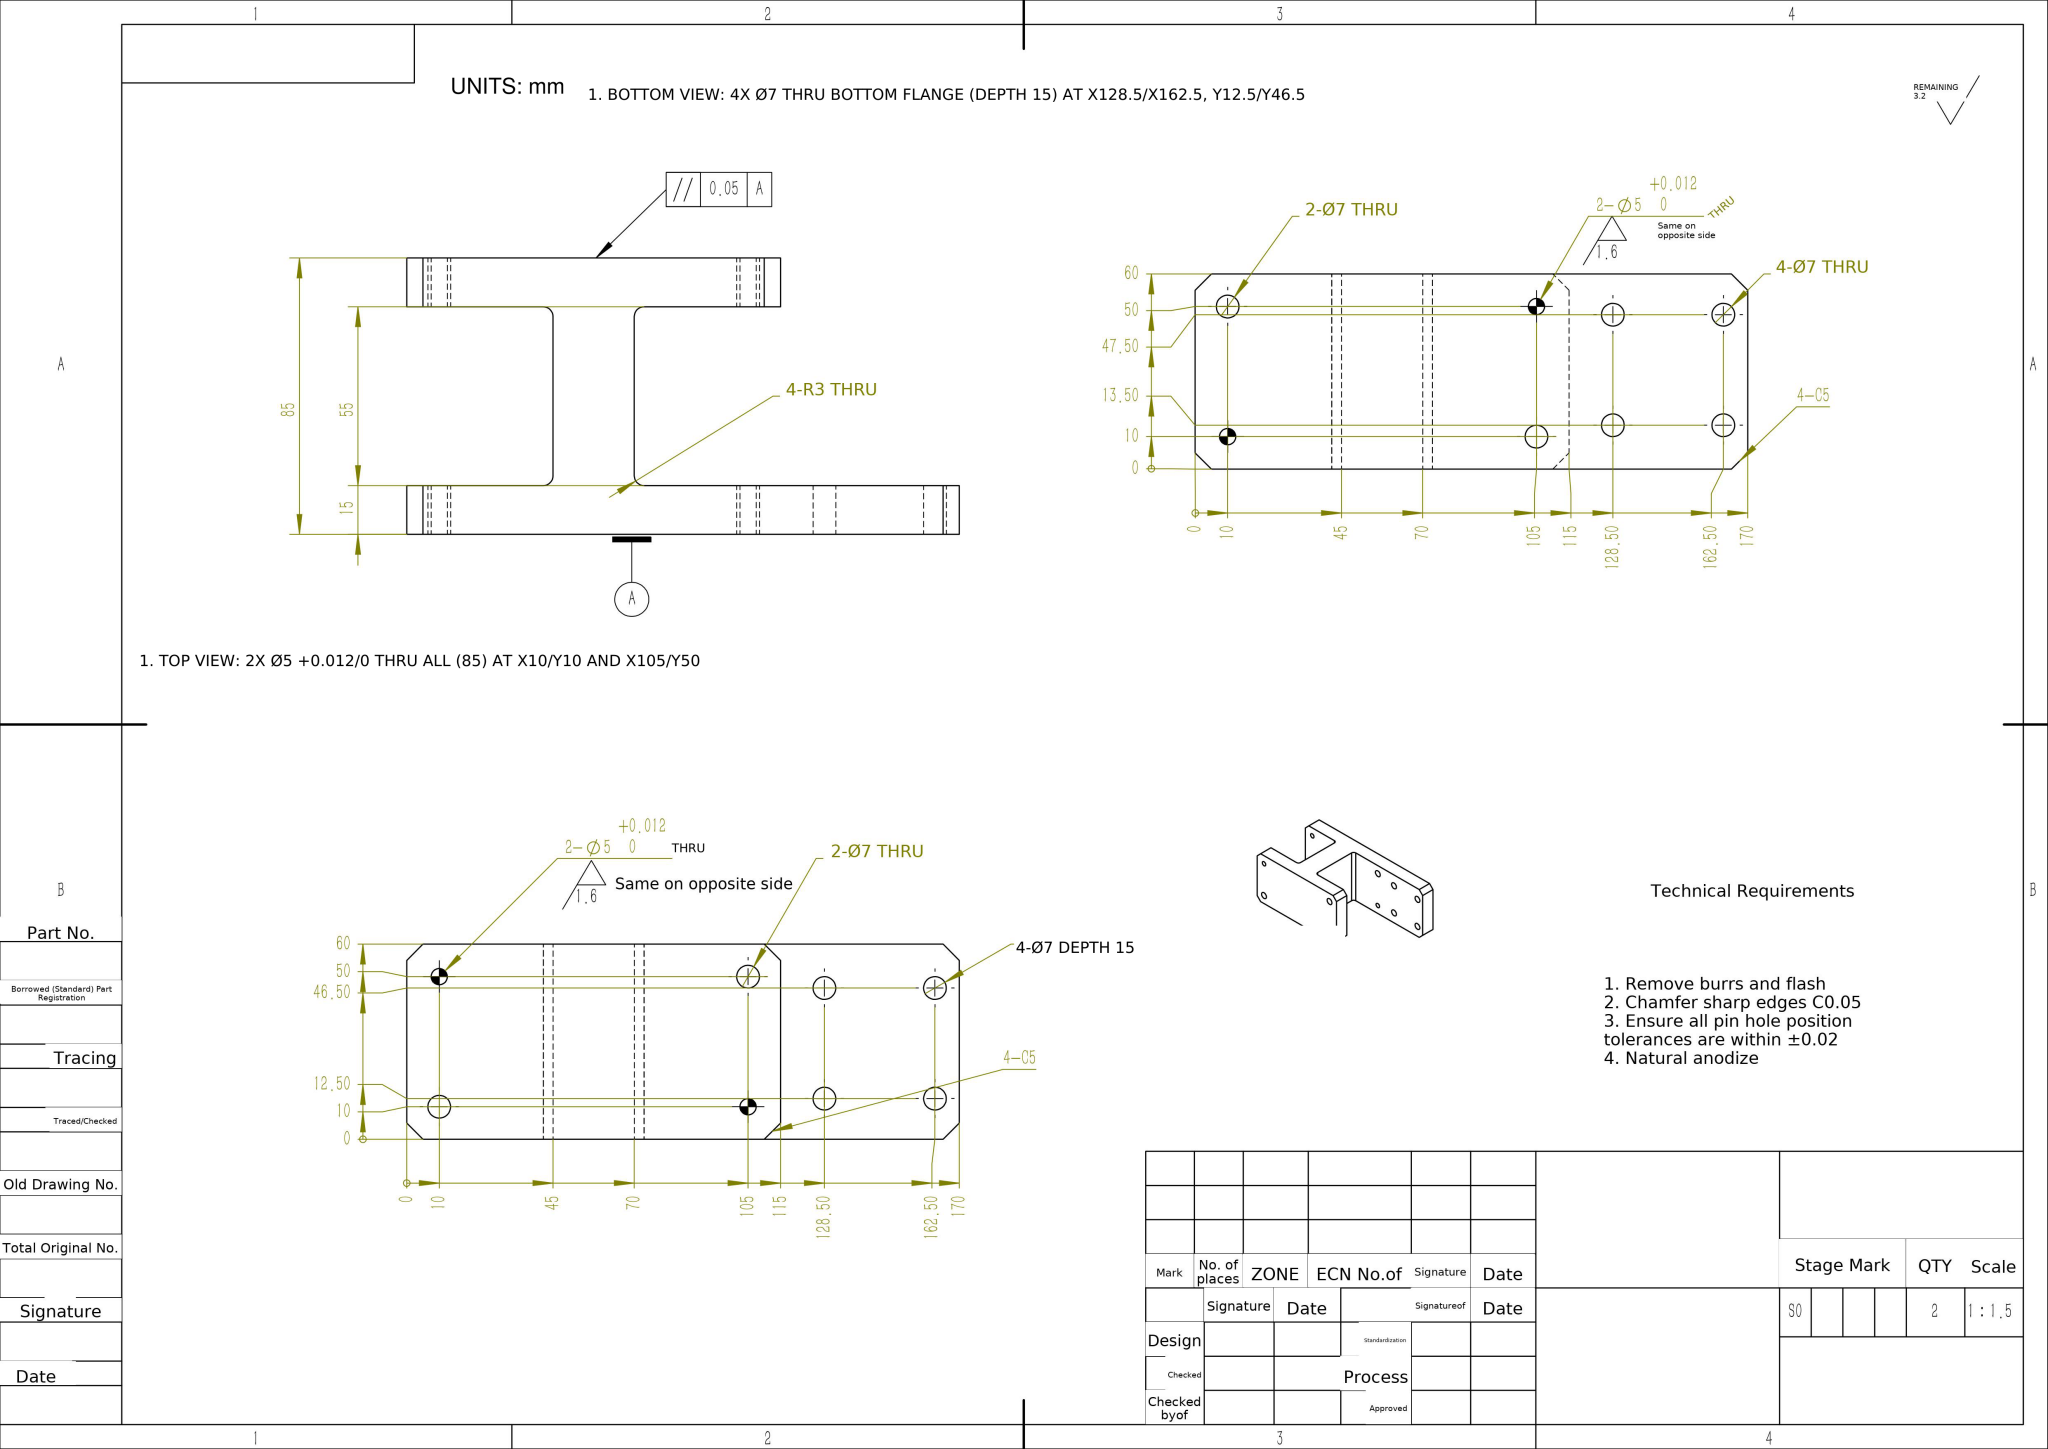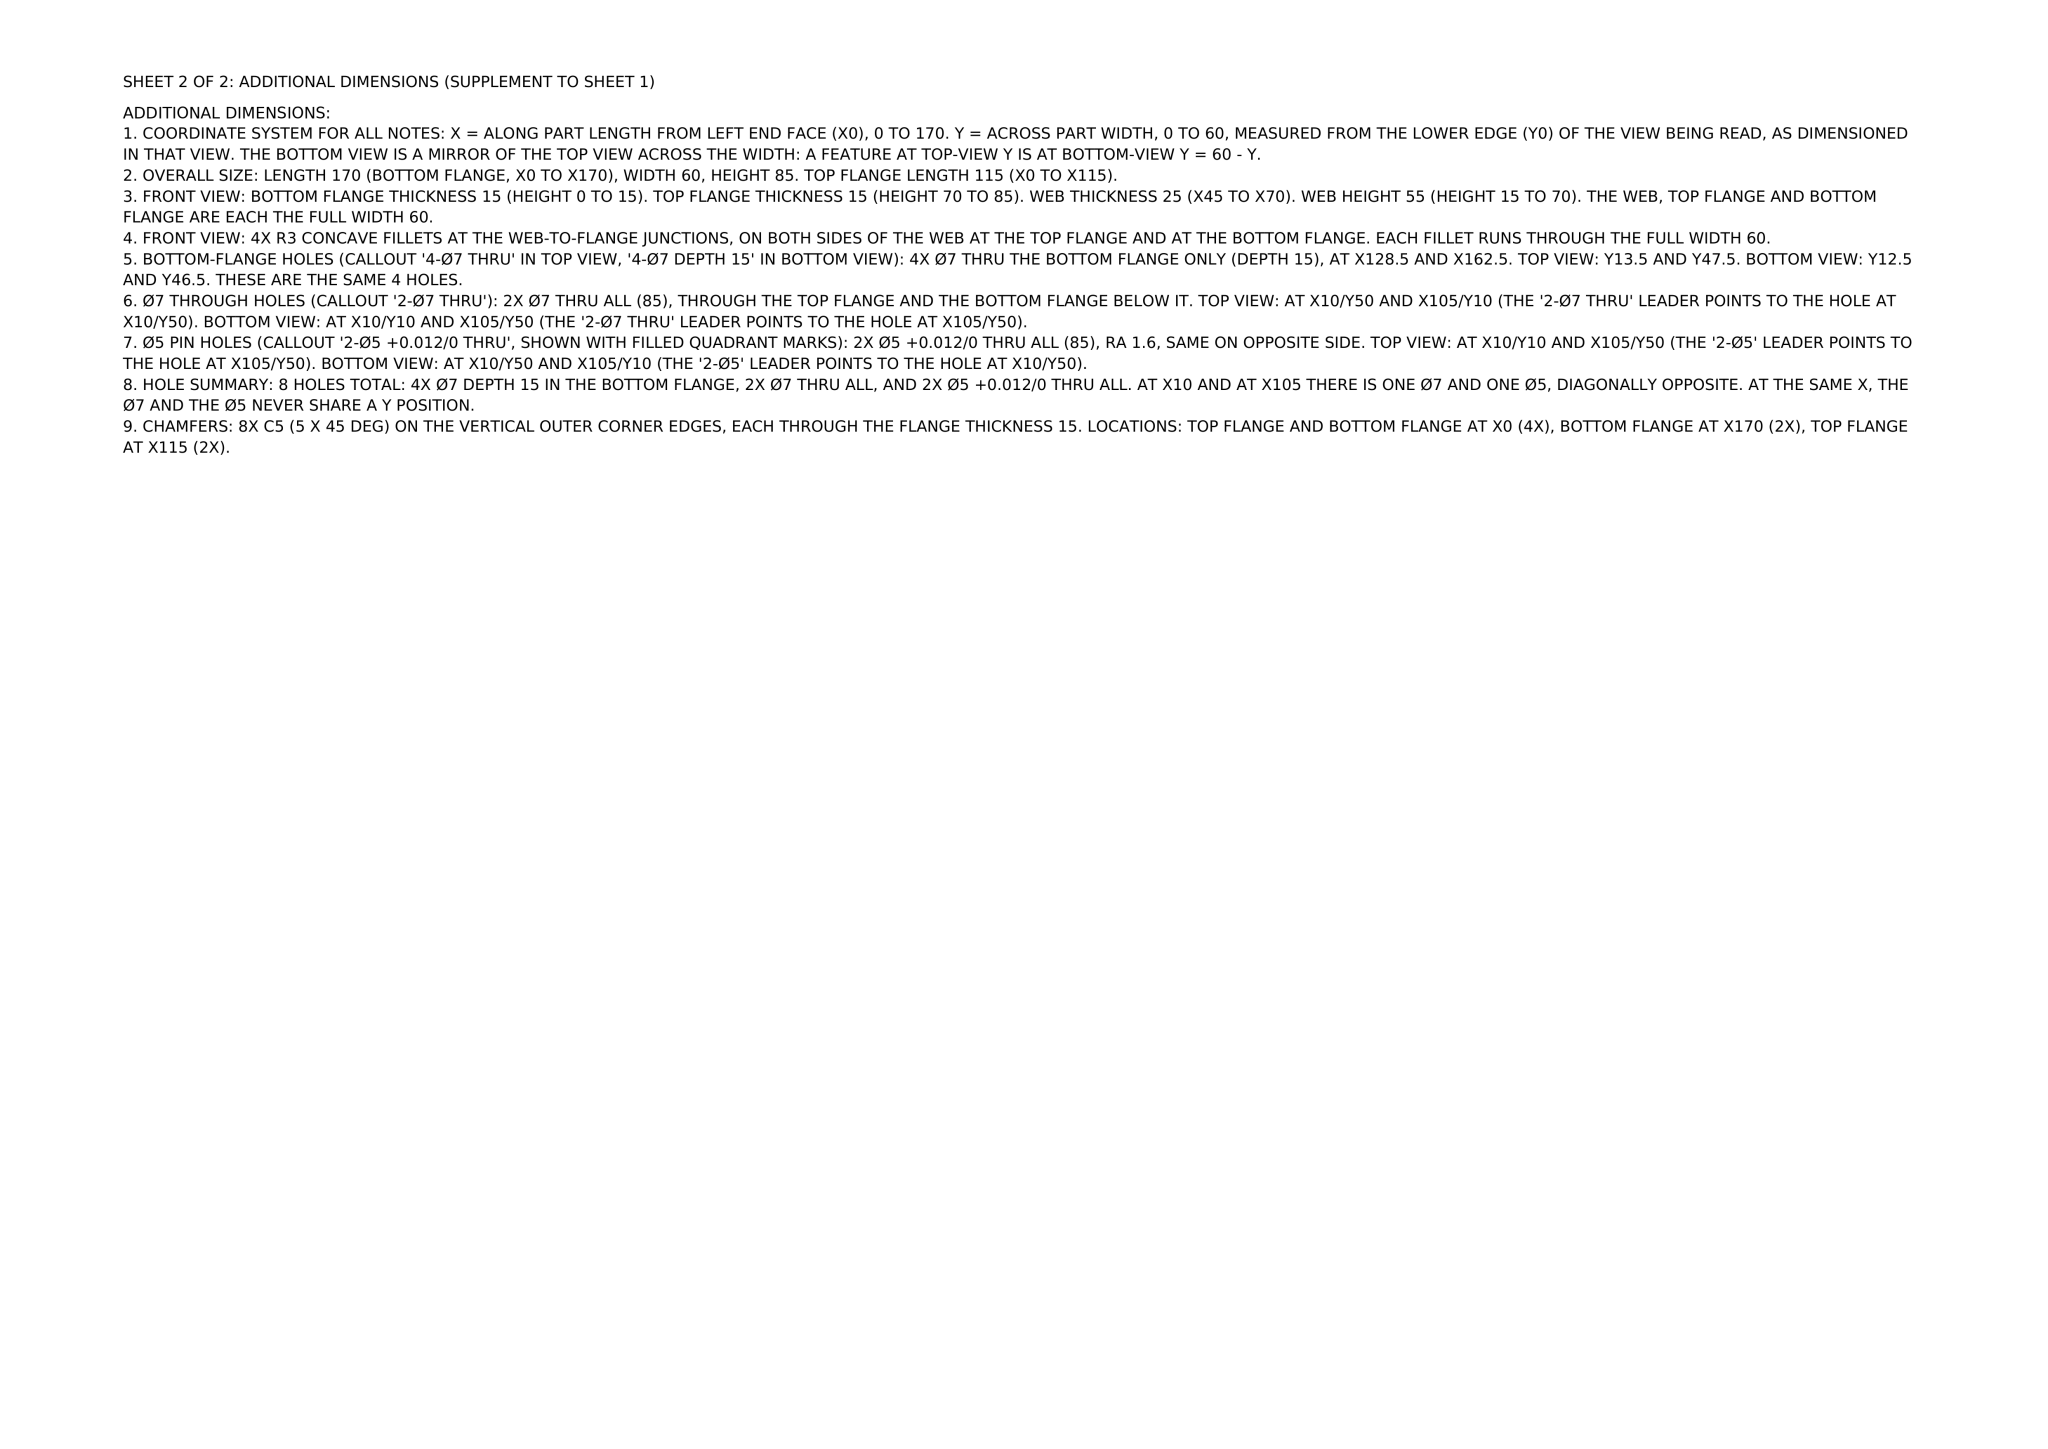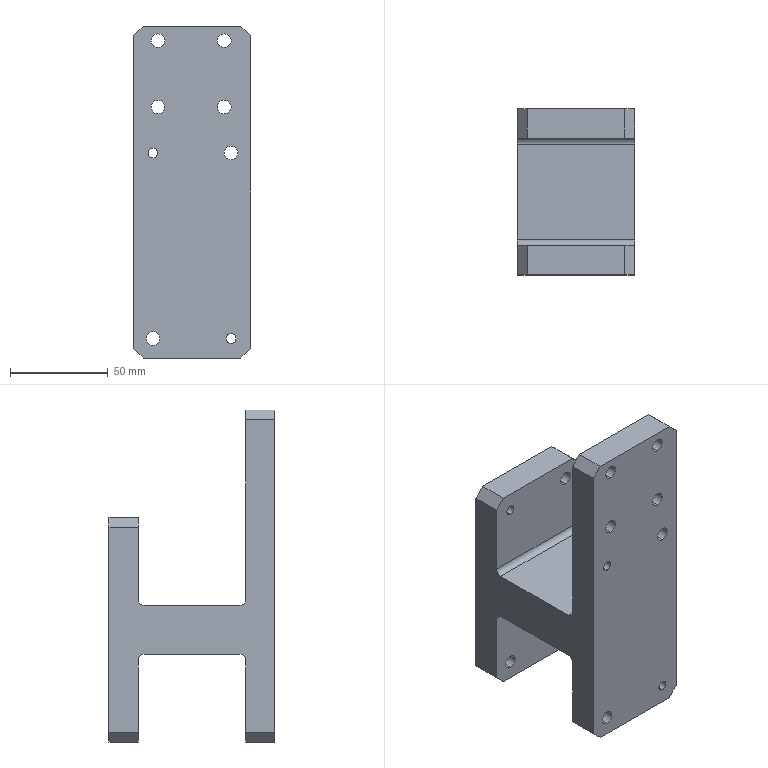Part | NX | mm | 1 solid | 50 faces | box 60 x 85 x 170 mm | volume 332167 mm3 | cylinder 28 | plane 22 | commonest cylinder face diameters 7 x16 5 x8 6 x4